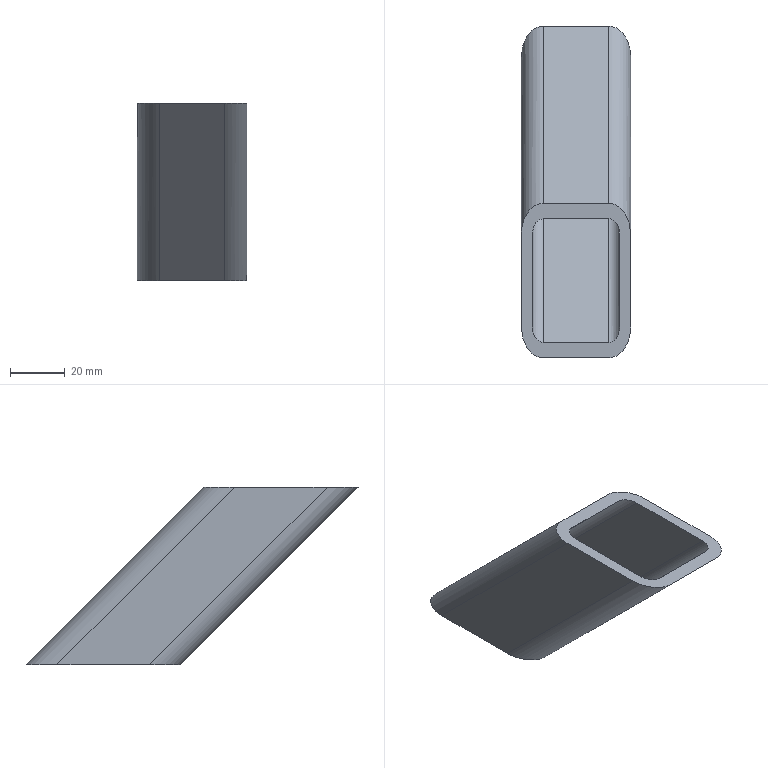Component | SolidWorks | 01-01Chassis-1_01-01-02ChassisWeldment2-1 | 1 solid | 18 faces | box 40 x 121.57 x 65 mm | volume 49161 mm3 | plane 10 | cylinder 8 | commonest cylinder face diameters 16 x4 8 x4 | material Q235
STEP:
#1=COLOUR_RGB('',0.7922,0.8196,0.9333);
#2=FILL_AREA_STYLE_COLOUR('',#1);
#3=FILL_AREA_STYLE('',(#2));
#4=SURFACE_STYLE_FILL_AREA(#3);
#5=SURFACE_SIDE_STYLE('',(#4));
#6=SURFACE_STYLE_USAGE(.BOTH.,#5);
#7=PRESENTATION_STYLE_ASSIGNMENT((#6));
#8=CARTESIAN_POINT('',(11.339,1.575,14.961));
#9=VERTEX_POINT('',#8);
#10=CARTESIAN_POINT('',(12.283,1.575,14.961));
#11=VERTEX_POINT('',#10);
#12=CARTESIAN_POINT('',(12.283,1.575,14.961));
#13=DIRECTION('',(1.,-0.,-0.));
#14=VECTOR('',#13,39.37);
#15=LINE('',#12,#14);
#16=EDGE_CURVE('',#9,#11,#15,.T.);
#17=ORIENTED_EDGE('',*,*,#16,.F.);
#18=CARTESIAN_POINT('',(11.339,-0.9843,17.52));
#19=VERTEX_POINT('',#18);
#20=CARTESIAN_POINT('',(11.339,1.892,14.643));
#21=DIRECTION('',(0.,-0.7071,0.7071));
#22=VECTOR('',#21,39.37);
#23=LINE('',#20,#22);
#24=EDGE_CURVE('',#9,#19,#23,.T.);
#25=ORIENTED_EDGE('',*,*,#24,.T.);
#26=CARTESIAN_POINT('',(12.283,-0.9843,17.52));
#27=VERTEX_POINT('',#26);
#28=CARTESIAN_POINT('',(12.283,-0.9843,17.52));
#29=DIRECTION('',(-1.,0.,0.));
#30=VECTOR('',#29,39.37);
#31=LINE('',#28,#30);
#32=EDGE_CURVE('',#27,#19,#31,.T.);
#33=ORIENTED_EDGE('',*,*,#32,.F.);
#34=CARTESIAN_POINT('',(12.283,1.892,14.643));
#35=DIRECTION('',(0.,-0.7071,0.7071));
#36=VECTOR('',#35,39.37);
#37=LINE('',#34,#36);
#38=EDGE_CURVE('',#11,#27,#37,.T.);
#39=ORIENTED_EDGE('',*,*,#38,.F.);
#40=EDGE_LOOP('',(#17,#25,#33,#39));
#41=FACE_OUTER_BOUND('',#40,.T.);
#42=CARTESIAN_POINT('',(12.283,1.892,14.643));
#43=DIRECTION('',(-0.,-0.7071,-0.7071));
#44=DIRECTION('',(-1.,0.,0.));
#45=AXIS2_PLACEMENT_3D('',#42,#43,#44);
#46=PLANE('',#45);
#47=ADVANCED_FACE('',(#41),#46,.F.);
#48=CARTESIAN_POINT('',(11.024,1.129,14.961));
#49=VERTEX_POINT('',#48);
#50=CARTESIAN_POINT('',(11.024,1.129,14.961));
#51=CARTESIAN_POINT('',(11.024,1.39,14.961));
#52=CARTESIAN_POINT('',(11.154,1.575,14.961));
#53=CARTESIAN_POINT('',(11.339,1.575,14.961));
#54=(BOUNDED_CURVE()B_SPLINE_CURVE(3,(#50,#51,#52,#53),.UNSPECIFIED.,.F.,.F.)B_SPLINE_CURVE_WITH_KNOTS((4,4),(1.571,3.142),.UNSPECIFIED.)CURVE()GEOMETRIC_REPRESENTATION_ITEM()RATIONAL_B_SPLINE_CURVE((1.,0.8047,0.8047,1.))REPRESENTATION_ITEM(''));
#55=EDGE_CURVE('',#49,#9,#54,.T.);
#56=ORIENTED_EDGE('',*,*,#55,.F.);
#57=CARTESIAN_POINT('',(11.024,-1.43,17.52));
#58=VERTEX_POINT('',#57);
#59=CARTESIAN_POINT('',(11.024,1.67,14.42));
#60=DIRECTION('',(0.,-0.7071,0.7071));
#61=VECTOR('',#60,39.37);
#62=LINE('',#59,#61);
#63=EDGE_CURVE('',#49,#58,#62,.T.);
#64=ORIENTED_EDGE('',*,*,#63,.T.);
#65=CARTESIAN_POINT('',(11.339,-0.9843,17.52));
#66=CARTESIAN_POINT('',(11.154,-0.9843,17.52));
#67=CARTESIAN_POINT('',(11.024,-1.169,17.52));
#68=CARTESIAN_POINT('',(11.024,-1.43,17.52));
#69=(BOUNDED_CURVE()B_SPLINE_CURVE(3,(#65,#66,#67,#68),.UNSPECIFIED.,.F.,.F.)B_SPLINE_CURVE_WITH_KNOTS((4,4),(3.142,4.712),.UNSPECIFIED.)CURVE()GEOMETRIC_REPRESENTATION_ITEM()RATIONAL_B_SPLINE_CURVE((1.,0.8047,0.8047,1.))REPRESENTATION_ITEM(''));
#70=EDGE_CURVE('',#19,#58,#69,.T.);
#71=ORIENTED_EDGE('',*,*,#70,.F.);
#72=ORIENTED_EDGE('',*,*,#24,.F.);
#73=EDGE_LOOP('',(#56,#64,#71,#72));
#74=FACE_OUTER_BOUND('',#73,.T.);
#75=CARTESIAN_POINT('',(11.339,1.67,14.42));
#76=DIRECTION('',(0.,-0.7071,0.7071));
#77=DIRECTION('',(-1.,0.,0.));
#78=AXIS2_PLACEMENT_3D('',#75,#76,#77);
#79=CYLINDRICAL_SURFACE('',#78,0.315);
#80=ADVANCED_FACE('',(#74),#79,.T.);
#81=CARTESIAN_POINT('',(11.024,-0.2069,14.961));
#82=VERTEX_POINT('',#81);
#83=CARTESIAN_POINT('',(11.024,2.686,14.961));
#84=DIRECTION('',(0.,1.,0.));
#85=VECTOR('',#84,39.37);
#86=LINE('',#83,#85);
#87=EDGE_CURVE('',#82,#49,#86,.T.);
#88=ORIENTED_EDGE('',*,*,#87,.F.);
#89=CARTESIAN_POINT('',(11.024,-2.766,17.52));
#90=VERTEX_POINT('',#89);
#91=CARTESIAN_POINT('',(11.024,1.001,13.752));
#92=DIRECTION('',(0.,-0.7071,0.7071));
#93=VECTOR('',#92,39.37);
#94=LINE('',#91,#93);
#95=EDGE_CURVE('',#82,#90,#94,.T.);
#96=ORIENTED_EDGE('',*,*,#95,.T.);
#97=CARTESIAN_POINT('',(11.024,2.686,17.52));
#98=DIRECTION('',(-0.,-1.,-0.));
#99=VECTOR('',#98,39.37);
#100=LINE('',#97,#99);
#101=EDGE_CURVE('',#58,#90,#100,.T.);
#102=ORIENTED_EDGE('',*,*,#101,.F.);
#103=ORIENTED_EDGE('',*,*,#63,.F.);
#104=EDGE_LOOP('',(#88,#96,#102,#103));
#105=FACE_OUTER_BOUND('',#104,.T.);
#106=CARTESIAN_POINT('',(11.024,1.001,13.752));
#107=DIRECTION('',(1.,-0.,-0.));
#108=DIRECTION('',(-0.,-0.7071,-0.7071));
#109=AXIS2_PLACEMENT_3D('',#106,#107,#108);
#110=PLANE('',#109);
#111=ADVANCED_FACE('',(#105),#110,.F.);
#112=CARTESIAN_POINT('',(11.339,-0.6523,14.961));
#113=VERTEX_POINT('',#112);
#114=CARTESIAN_POINT('',(11.339,-0.6523,14.961));
#115=CARTESIAN_POINT('',(11.154,-0.6523,14.961));
#116=CARTESIAN_POINT('',(11.024,-0.4678,14.961));
#117=CARTESIAN_POINT('',(11.024,-0.2069,14.961));
#118=(BOUNDED_CURVE()B_SPLINE_CURVE(3,(#114,#115,#116,#117),.UNSPECIFIED.,.F.,.F.)B_SPLINE_CURVE_WITH_KNOTS((4,4),(0.,1.571),.UNSPECIFIED.)CURVE()GEOMETRIC_REPRESENTATION_ITEM()RATIONAL_B_SPLINE_CURVE((1.,0.8047,0.8047,1.))REPRESENTATION_ITEM(''));
#119=EDGE_CURVE('',#113,#82,#118,.T.);
#120=ORIENTED_EDGE('',*,*,#119,.F.);
#121=CARTESIAN_POINT('',(11.339,-3.211,17.52));
#122=VERTEX_POINT('',#121);
#123=CARTESIAN_POINT('',(11.339,0.7788,13.53));
#124=DIRECTION('',(0.,-0.7071,0.7071));
#125=VECTOR('',#124,39.37);
#126=LINE('',#123,#125);
#127=EDGE_CURVE('',#113,#122,#126,.T.);
#128=ORIENTED_EDGE('',*,*,#127,.T.);
#129=CARTESIAN_POINT('',(11.024,-2.766,17.52));
#130=CARTESIAN_POINT('',(11.024,-3.027,17.52));
#131=CARTESIAN_POINT('',(11.154,-3.211,17.52));
#132=CARTESIAN_POINT('',(11.339,-3.211,17.52));
#133=(BOUNDED_CURVE()B_SPLINE_CURVE(3,(#129,#130,#131,#132),.UNSPECIFIED.,.F.,.F.)B_SPLINE_CURVE_WITH_KNOTS((4,4),(4.712,6.283),.UNSPECIFIED.)CURVE()GEOMETRIC_REPRESENTATION_ITEM()RATIONAL_B_SPLINE_CURVE((1.,0.8047,0.8047,1.))REPRESENTATION_ITEM(''));
#134=EDGE_CURVE('',#90,#122,#133,.T.);
#135=ORIENTED_EDGE('',*,*,#134,.F.);
#136=ORIENTED_EDGE('',*,*,#95,.F.);
#137=EDGE_LOOP('',(#120,#128,#135,#136));
#138=FACE_OUTER_BOUND('',#137,.T.);
#139=CARTESIAN_POINT('',(11.339,1.001,13.752));
#140=DIRECTION('',(0.,-0.7071,0.7071));
#141=DIRECTION('',(-1.,0.,0.));
#142=AXIS2_PLACEMENT_3D('',#139,#140,#141);
#143=CYLINDRICAL_SURFACE('',#142,0.315);
#144=ADVANCED_FACE('',(#138),#143,.T.);
#145=CARTESIAN_POINT('',(12.283,-0.6523,14.961));
#146=VERTEX_POINT('',#145);
#147=CARTESIAN_POINT('',(11.339,-0.6523,14.961));
#148=DIRECTION('',(-1.,0.,0.));
#149=VECTOR('',#148,39.37);
#150=LINE('',#147,#149);
#151=EDGE_CURVE('',#146,#113,#150,.T.);
#152=ORIENTED_EDGE('',*,*,#151,.F.);
#153=CARTESIAN_POINT('',(12.283,-3.211,17.52));
#154=VERTEX_POINT('',#153);
#155=CARTESIAN_POINT('',(12.283,0.7788,13.53));
#156=DIRECTION('',(0.,-0.7071,0.7071));
#157=VECTOR('',#156,39.37);
#158=LINE('',#155,#157);
#159=EDGE_CURVE('',#146,#154,#158,.T.);
#160=ORIENTED_EDGE('',*,*,#159,.T.);
#161=CARTESIAN_POINT('',(11.339,-3.211,17.52));
#162=DIRECTION('',(1.,-0.,-0.));
#163=VECTOR('',#162,39.37);
#164=LINE('',#161,#163);
#165=EDGE_CURVE('',#122,#154,#164,.T.);
#166=ORIENTED_EDGE('',*,*,#165,.F.);
#167=ORIENTED_EDGE('',*,*,#127,.F.);
#168=EDGE_LOOP('',(#152,#160,#166,#167));
#169=FACE_OUTER_BOUND('',#168,.T.);
#170=CARTESIAN_POINT('',(11.339,0.7788,13.53));
#171=DIRECTION('',(0.,0.7071,0.7071));
#172=DIRECTION('',(1.,-0.,-0.));
#173=AXIS2_PLACEMENT_3D('',#170,#171,#172);
#174=PLANE('',#173);
#175=ADVANCED_FACE('',(#169),#174,.F.);
#176=CARTESIAN_POINT('',(12.598,-0.2069,14.961));
#177=VERTEX_POINT('',#176);
#178=CARTESIAN_POINT('',(12.598,-0.2069,14.961));
#179=CARTESIAN_POINT('',(12.598,-0.4678,14.961));
#180=CARTESIAN_POINT('',(12.468,-0.6523,14.961));
#181=CARTESIAN_POINT('',(12.283,-0.6523,14.961));
#182=(BOUNDED_CURVE()B_SPLINE_CURVE(3,(#178,#179,#180,#181),.UNSPECIFIED.,.F.,.F.)B_SPLINE_CURVE_WITH_KNOTS((4,4),(4.712,6.283),.UNSPECIFIED.)CURVE()GEOMETRIC_REPRESENTATION_ITEM()RATIONAL_B_SPLINE_CURVE((1.,0.8047,0.8047,1.))REPRESENTATION_ITEM(''));
#183=EDGE_CURVE('',#177,#146,#182,.T.);
#184=ORIENTED_EDGE('',*,*,#183,.F.);
#185=CARTESIAN_POINT('',(12.598,-2.766,17.52));
#186=VERTEX_POINT('',#185);
#187=CARTESIAN_POINT('',(12.598,1.001,13.752));
#188=DIRECTION('',(0.,-0.7071,0.7071));
#189=VECTOR('',#188,39.37);
#190=LINE('',#187,#189);
#191=EDGE_CURVE('',#177,#186,#190,.T.);
#192=ORIENTED_EDGE('',*,*,#191,.T.);
#193=CARTESIAN_POINT('',(12.283,-3.211,17.52));
#194=CARTESIAN_POINT('',(12.468,-3.211,17.52));
#195=CARTESIAN_POINT('',(12.598,-3.027,17.52));
#196=CARTESIAN_POINT('',(12.598,-2.766,17.52));
#197=(BOUNDED_CURVE()B_SPLINE_CURVE(3,(#193,#194,#195,#196),.UNSPECIFIED.,.F.,.F.)B_SPLINE_CURVE_WITH_KNOTS((4,4),(0.,1.571),.UNSPECIFIED.)CURVE()GEOMETRIC_REPRESENTATION_ITEM()RATIONAL_B_SPLINE_CURVE((1.,0.8047,0.8047,1.))REPRESENTATION_ITEM(''));
#198=EDGE_CURVE('',#154,#186,#197,.T.);
#199=ORIENTED_EDGE('',*,*,#198,.F.);
#200=ORIENTED_EDGE('',*,*,#159,.F.);
#201=EDGE_LOOP('',(#184,#192,#199,#200));
#202=FACE_OUTER_BOUND('',#201,.T.);
#203=CARTESIAN_POINT('',(12.283,1.001,13.752));
#204=DIRECTION('',(0.,-0.7071,0.7071));
#205=DIRECTION('',(-1.,0.,0.));
#206=AXIS2_PLACEMENT_3D('',#203,#204,#205);
#207=CYLINDRICAL_SURFACE('',#206,0.315);
#208=ADVANCED_FACE('',(#202),#207,.T.);
#209=CARTESIAN_POINT('',(12.598,1.129,14.961));
#210=VERTEX_POINT('',#209);
#211=CARTESIAN_POINT('',(12.598,2.686,14.961));
#212=DIRECTION('',(0.,1.,0.));
#213=VECTOR('',#212,39.37);
#214=LINE('',#211,#213);
#215=EDGE_CURVE('',#177,#210,#214,.T.);
#216=ORIENTED_EDGE('',*,*,#215,.T.);
#217=CARTESIAN_POINT('',(12.598,-1.43,17.52));
#218=VERTEX_POINT('',#217);
#219=CARTESIAN_POINT('',(12.598,1.67,14.42));
#220=DIRECTION('',(0.,-0.7071,0.7071));
#221=VECTOR('',#220,39.37);
#222=LINE('',#219,#221);
#223=EDGE_CURVE('',#210,#218,#222,.T.);
#224=ORIENTED_EDGE('',*,*,#223,.T.);
#225=CARTESIAN_POINT('',(12.598,2.686,17.52));
#226=DIRECTION('',(-0.,-1.,-0.));
#227=VECTOR('',#226,39.37);
#228=LINE('',#225,#227);
#229=EDGE_CURVE('',#218,#186,#228,.T.);
#230=ORIENTED_EDGE('',*,*,#229,.T.);
#231=ORIENTED_EDGE('',*,*,#191,.F.);
#232=EDGE_LOOP('',(#216,#224,#230,#231));
#233=FACE_OUTER_BOUND('',#232,.T.);
#234=CARTESIAN_POINT('',(12.598,1.67,14.42));
#235=DIRECTION('',(-1.,0.,0.));
#236=DIRECTION('',(0.,0.7071,0.7071));
#237=AXIS2_PLACEMENT_3D('',#234,#235,#236);
#238=PLANE('',#237);
#239=ADVANCED_FACE('',(#233),#238,.F.);
#240=CARTESIAN_POINT('',(12.283,1.575,14.961));
#241=CARTESIAN_POINT('',(12.468,1.575,14.961));
#242=CARTESIAN_POINT('',(12.598,1.39,14.961));
#243=CARTESIAN_POINT('',(12.598,1.129,14.961));
#244=(BOUNDED_CURVE()B_SPLINE_CURVE(3,(#240,#241,#242,#243),.UNSPECIFIED.,.F.,.F.)B_SPLINE_CURVE_WITH_KNOTS((4,4),(3.142,4.712),.UNSPECIFIED.)CURVE()GEOMETRIC_REPRESENTATION_ITEM()RATIONAL_B_SPLINE_CURVE((1.,0.8047,0.8047,1.))REPRESENTATION_ITEM(''));
#245=EDGE_CURVE('',#11,#210,#244,.T.);
#246=ORIENTED_EDGE('',*,*,#245,.F.);
#247=ORIENTED_EDGE('',*,*,#38,.T.);
#248=CARTESIAN_POINT('',(12.598,-1.43,17.52));
#249=CARTESIAN_POINT('',(12.598,-1.169,17.52));
#250=CARTESIAN_POINT('',(12.468,-0.9843,17.52));
#251=CARTESIAN_POINT('',(12.283,-0.9843,17.52));
#252=(BOUNDED_CURVE()B_SPLINE_CURVE(3,(#248,#249,#250,#251),.UNSPECIFIED.,.F.,.F.)B_SPLINE_CURVE_WITH_KNOTS((4,4),(1.571,3.142),.UNSPECIFIED.)CURVE()GEOMETRIC_REPRESENTATION_ITEM()RATIONAL_B_SPLINE_CURVE((1.,0.8047,0.8047,1.))REPRESENTATION_ITEM(''));
#253=EDGE_CURVE('',#218,#27,#252,.T.);
#254=ORIENTED_EDGE('',*,*,#253,.F.);
#255=ORIENTED_EDGE('',*,*,#223,.F.);
#256=EDGE_LOOP('',(#246,#247,#254,#255));
#257=FACE_OUTER_BOUND('',#256,.T.);
#258=CARTESIAN_POINT('',(12.283,1.67,14.42));
#259=DIRECTION('',(0.,-0.7071,0.7071));
#260=DIRECTION('',(-1.,0.,0.));
#261=AXIS2_PLACEMENT_3D('',#258,#259,#260);
#262=CYLINDRICAL_SURFACE('',#261,0.315);
#263=ADVANCED_FACE('',(#257),#262,.T.);
#264=CARTESIAN_POINT('',(11.339,-2.989,17.52));
#265=VERTEX_POINT('',#264);
#266=CARTESIAN_POINT('',(12.283,-2.989,17.52));
#267=VERTEX_POINT('',#266);
#268=CARTESIAN_POINT('',(11.339,-2.989,17.52));
#269=DIRECTION('',(1.,-0.,-0.));
#270=VECTOR('',#269,39.37);
#271=LINE('',#268,#270);
#272=EDGE_CURVE('',#265,#267,#271,.T.);
#273=ORIENTED_EDGE('',*,*,#272,.F.);
#274=CARTESIAN_POINT('',(11.181,-2.766,17.52));
#275=VERTEX_POINT('',#274);
#276=CARTESIAN_POINT('',(11.181,-2.766,17.52));
#277=CARTESIAN_POINT('',(11.181,-2.896,17.52));
#278=CARTESIAN_POINT('',(11.246,-2.989,17.52));
#279=CARTESIAN_POINT('',(11.339,-2.989,17.52));
#280=(BOUNDED_CURVE()B_SPLINE_CURVE(3,(#276,#277,#278,#279),.UNSPECIFIED.,.F.,.F.)B_SPLINE_CURVE_WITH_KNOTS((4,4),(4.712,6.283),.UNSPECIFIED.)CURVE()GEOMETRIC_REPRESENTATION_ITEM()RATIONAL_B_SPLINE_CURVE((1.,0.8047,0.8047,1.))REPRESENTATION_ITEM(''));
#281=EDGE_CURVE('',#275,#265,#280,.T.);
#282=ORIENTED_EDGE('',*,*,#281,.F.);
#283=CARTESIAN_POINT('',(11.181,-1.43,17.52));
#284=VERTEX_POINT('',#283);
#285=CARTESIAN_POINT('',(11.181,1.001,17.52));
#286=DIRECTION('',(-0.,-1.,-0.));
#287=VECTOR('',#286,39.37);
#288=LINE('',#285,#287);
#289=EDGE_CURVE('',#284,#275,#288,.T.);
#290=ORIENTED_EDGE('',*,*,#289,.F.);
#291=CARTESIAN_POINT('',(11.339,-1.207,17.52));
#292=VERTEX_POINT('',#291);
#293=CARTESIAN_POINT('',(11.339,-1.207,17.52));
#294=CARTESIAN_POINT('',(11.246,-1.207,17.52));
#295=CARTESIAN_POINT('',(11.181,-1.299,17.52));
#296=CARTESIAN_POINT('',(11.181,-1.43,17.52));
#297=(BOUNDED_CURVE()B_SPLINE_CURVE(3,(#293,#294,#295,#296),.UNSPECIFIED.,.F.,.F.)B_SPLINE_CURVE_WITH_KNOTS((4,4),(3.142,4.712),.UNSPECIFIED.)CURVE()GEOMETRIC_REPRESENTATION_ITEM()RATIONAL_B_SPLINE_CURVE((1.,0.8047,0.8047,1.))REPRESENTATION_ITEM(''));
#298=EDGE_CURVE('',#292,#284,#297,.T.);
#299=ORIENTED_EDGE('',*,*,#298,.F.);
#300=CARTESIAN_POINT('',(12.283,-1.207,17.52));
#301=VERTEX_POINT('',#300);
#302=CARTESIAN_POINT('',(12.283,-1.207,17.52));
#303=DIRECTION('',(-1.,0.,0.));
#304=VECTOR('',#303,39.37);
#305=LINE('',#302,#304);
#306=EDGE_CURVE('',#301,#292,#305,.T.);
#307=ORIENTED_EDGE('',*,*,#306,.F.);
#308=CARTESIAN_POINT('',(12.441,-1.43,17.52));
#309=VERTEX_POINT('',#308);
#310=CARTESIAN_POINT('',(12.441,-1.43,17.52));
#311=CARTESIAN_POINT('',(12.441,-1.299,17.52));
#312=CARTESIAN_POINT('',(12.376,-1.207,17.52));
#313=CARTESIAN_POINT('',(12.283,-1.207,17.52));
#314=(BOUNDED_CURVE()B_SPLINE_CURVE(3,(#310,#311,#312,#313),.UNSPECIFIED.,.F.,.F.)B_SPLINE_CURVE_WITH_KNOTS((4,4),(1.571,3.142),.UNSPECIFIED.)CURVE()GEOMETRIC_REPRESENTATION_ITEM()RATIONAL_B_SPLINE_CURVE((1.,0.8047,0.8047,1.))REPRESENTATION_ITEM(''));
#315=EDGE_CURVE('',#309,#301,#314,.T.);
#316=ORIENTED_EDGE('',*,*,#315,.F.);
#317=CARTESIAN_POINT('',(12.441,-2.766,17.52));
#318=VERTEX_POINT('',#317);
#319=CARTESIAN_POINT('',(12.441,1.67,17.52));
#320=DIRECTION('',(0.,1.,0.));
#321=VECTOR('',#320,39.37);
#322=LINE('',#319,#321);
#323=EDGE_CURVE('',#318,#309,#322,.T.);
#324=ORIENTED_EDGE('',*,*,#323,.F.);
#325=CARTESIAN_POINT('',(12.283,-2.989,17.52));
#326=CARTESIAN_POINT('',(12.376,-2.989,17.52));
#327=CARTESIAN_POINT('',(12.441,-2.896,17.52));
#328=CARTESIAN_POINT('',(12.441,-2.766,17.52));
#329=(BOUNDED_CURVE()B_SPLINE_CURVE(3,(#325,#326,#327,#328),.UNSPECIFIED.,.F.,.F.)B_SPLINE_CURVE_WITH_KNOTS((4,4),(0.,1.571),.UNSPECIFIED.)CURVE()GEOMETRIC_REPRESENTATION_ITEM()RATIONAL_B_SPLINE_CURVE((1.,0.8047,0.8047,1.))REPRESENTATION_ITEM(''));
#330=EDGE_CURVE('',#267,#318,#329,.T.);
#331=ORIENTED_EDGE('',*,*,#330,.F.);
#332=EDGE_LOOP('',(#273,#282,#290,#299,#307,#316,#324,#331));
#333=FACE_BOUND('',#332,.T.);
#334=ORIENTED_EDGE('',*,*,#198,.T.);
#335=ORIENTED_EDGE('',*,*,#229,.F.);
#336=ORIENTED_EDGE('',*,*,#253,.T.);
#337=ORIENTED_EDGE('',*,*,#32,.T.);
#338=ORIENTED_EDGE('',*,*,#70,.T.);
#339=ORIENTED_EDGE('',*,*,#101,.T.);
#340=ORIENTED_EDGE('',*,*,#134,.T.);
#341=ORIENTED_EDGE('',*,*,#165,.T.);
#342=EDGE_LOOP('',(#334,#335,#336,#337,#338,#339,#340,#341));
#343=FACE_OUTER_BOUND('',#342,.T.);
#344=CARTESIAN_POINT('',(11.024,2.686,17.52));
#345=DIRECTION('',(0.,-0.,1.));
#346=DIRECTION('',(-0.,-1.,-0.));
#347=AXIS2_PLACEMENT_3D('',#344,#345,#346);
#348=PLANE('',#347);
#349=ADVANCED_FACE('',(#333,#343),#348,.T.);
#350=CARTESIAN_POINT('',(12.441,1.129,14.961));
#351=VERTEX_POINT('',#350);
#352=CARTESIAN_POINT('',(12.441,-0.2069,14.961));
#353=VERTEX_POINT('',#352);
#354=CARTESIAN_POINT('',(12.441,1.67,14.961));
#355=DIRECTION('',(-0.,-1.,-0.));
#356=VECTOR('',#355,39.37);
#357=LINE('',#354,#356);
#358=EDGE_CURVE('',#351,#353,#357,.T.);
#359=ORIENTED_EDGE('',*,*,#358,.F.);
#360=CARTESIAN_POINT('',(12.283,1.352,14.961));
#361=VERTEX_POINT('',#360);
#362=CARTESIAN_POINT('',(12.283,1.352,14.961));
#363=CARTESIAN_POINT('',(12.376,1.352,14.961));
#364=CARTESIAN_POINT('',(12.441,1.26,14.961));
#365=CARTESIAN_POINT('',(12.441,1.129,14.961));
#366=(BOUNDED_CURVE()B_SPLINE_CURVE(3,(#362,#363,#364,#365),.UNSPECIFIED.,.F.,.F.)B_SPLINE_CURVE_WITH_KNOTS((4,4),(3.142,4.712),.UNSPECIFIED.)CURVE()GEOMETRIC_REPRESENTATION_ITEM()RATIONAL_B_SPLINE_CURVE((1.,0.8047,0.8047,1.))REPRESENTATION_ITEM(''));
#367=EDGE_CURVE('',#361,#351,#366,.T.);
#368=ORIENTED_EDGE('',*,*,#367,.F.);
#369=CARTESIAN_POINT('',(11.339,1.352,14.961));
#370=VERTEX_POINT('',#369);
#371=CARTESIAN_POINT('',(12.283,1.352,14.961));
#372=DIRECTION('',(1.,-0.,-0.));
#373=VECTOR('',#372,39.37);
#374=LINE('',#371,#373);
#375=EDGE_CURVE('',#370,#361,#374,.T.);
#376=ORIENTED_EDGE('',*,*,#375,.F.);
#377=CARTESIAN_POINT('',(11.181,1.129,14.961));
#378=VERTEX_POINT('',#377);
#379=CARTESIAN_POINT('',(11.181,1.129,14.961));
#380=CARTESIAN_POINT('',(11.181,1.26,14.961));
#381=CARTESIAN_POINT('',(11.246,1.352,14.961));
#382=CARTESIAN_POINT('',(11.339,1.352,14.961));
#383=(BOUNDED_CURVE()B_SPLINE_CURVE(3,(#379,#380,#381,#382),.UNSPECIFIED.,.F.,.F.)B_SPLINE_CURVE_WITH_KNOTS((4,4),(1.571,3.142),.UNSPECIFIED.)CURVE()GEOMETRIC_REPRESENTATION_ITEM()RATIONAL_B_SPLINE_CURVE((1.,0.8047,0.8047,1.))REPRESENTATION_ITEM(''));
#384=EDGE_CURVE('',#378,#370,#383,.T.);
#385=ORIENTED_EDGE('',*,*,#384,.F.);
#386=CARTESIAN_POINT('',(11.181,-0.2069,14.961));
#387=VERTEX_POINT('',#386);
#388=CARTESIAN_POINT('',(11.181,1.001,14.961));
#389=DIRECTION('',(0.,1.,0.));
#390=VECTOR('',#389,39.37);
#391=LINE('',#388,#390);
#392=EDGE_CURVE('',#387,#378,#391,.T.);
#393=ORIENTED_EDGE('',*,*,#392,.F.);
#394=CARTESIAN_POINT('',(11.339,-0.4296,14.961));
#395=VERTEX_POINT('',#394);
#396=CARTESIAN_POINT('',(11.339,-0.4296,14.961));
#397=CARTESIAN_POINT('',(11.246,-0.4296,14.961));
#398=CARTESIAN_POINT('',(11.181,-0.3373,14.961));
#399=CARTESIAN_POINT('',(11.181,-0.2069,14.961));
#400=(BOUNDED_CURVE()B_SPLINE_CURVE(3,(#396,#397,#398,#399),.UNSPECIFIED.,.F.,.T.)B_SPLINE_CURVE_WITH_KNOTS((4,4),(0.,1.571),.UNSPECIFIED.)CURVE()GEOMETRIC_REPRESENTATION_ITEM()RATIONAL_B_SPLINE_CURVE((1.,0.8047,0.8047,1.))REPRESENTATION_ITEM(''));
#401=EDGE_CURVE('',#395,#387,#400,.T.);
#402=ORIENTED_EDGE('',*,*,#401,.F.);
#403=CARTESIAN_POINT('',(12.283,-0.4296,14.961));
#404=VERTEX_POINT('',#403);
#405=CARTESIAN_POINT('',(11.339,-0.4296,14.961));
#406=DIRECTION('',(-1.,0.,0.));
#407=VECTOR('',#406,39.37);
#408=LINE('',#405,#407);
#409=EDGE_CURVE('',#404,#395,#408,.T.);
#410=ORIENTED_EDGE('',*,*,#409,.F.);
#411=CARTESIAN_POINT('',(12.441,-0.2069,14.961));
#412=CARTESIAN_POINT('',(12.441,-0.3373,14.961));
#413=CARTESIAN_POINT('',(12.376,-0.4296,14.961));
#414=CARTESIAN_POINT('',(12.283,-0.4296,14.961));
#415=(BOUNDED_CURVE()B_SPLINE_CURVE(3,(#411,#412,#413,#414),.UNSPECIFIED.,.F.,.F.)B_SPLINE_CURVE_WITH_KNOTS((4,4),(4.712,6.283),.UNSPECIFIED.)CURVE()GEOMETRIC_REPRESENTATION_ITEM()RATIONAL_B_SPLINE_CURVE((1.,0.8047,0.8047,1.))REPRESENTATION_ITEM(''));
#416=EDGE_CURVE('',#353,#404,#415,.T.);
#417=ORIENTED_EDGE('',*,*,#416,.F.);
#418=EDGE_LOOP('',(#359,#368,#376,#385,#393,#402,#410,#417));
#419=FACE_BOUND('',#418,.T.);
#420=ORIENTED_EDGE('',*,*,#183,.T.);
#421=ORIENTED_EDGE('',*,*,#151,.T.);
#422=ORIENTED_EDGE('',*,*,#119,.T.);
#423=ORIENTED_EDGE('',*,*,#87,.T.);
#424=ORIENTED_EDGE('',*,*,#55,.T.);
#425=ORIENTED_EDGE('',*,*,#16,.T.);
#426=ORIENTED_EDGE('',*,*,#245,.T.);
#427=ORIENTED_EDGE('',*,*,#215,.F.);
#428=EDGE_LOOP('',(#420,#421,#422,#423,#424,#425,#426,#427));
#429=FACE_OUTER_BOUND('',#428,.T.);
#430=CARTESIAN_POINT('',(11.024,2.686,14.961));
#431=DIRECTION('',(-0.,0.,-1.));
#432=DIRECTION('',(0.,1.,0.));
#433=AXIS2_PLACEMENT_3D('',#430,#431,#432);
#434=PLANE('',#433);
#435=ADVANCED_FACE('',(#419,#429),#434,.T.);
#436=CARTESIAN_POINT('',(12.441,1.001,13.752));
#437=DIRECTION('',(0.,-0.7071,0.7071));
#438=VECTOR('',#437,39.37);
#439=LINE('',#436,#438);
#440=EDGE_CURVE('',#353,#318,#439,.T.);
#441=ORIENTED_EDGE('',*,*,#440,.F.);
#442=ORIENTED_EDGE('',*,*,#416,.T.);
#443=CARTESIAN_POINT('',(12.283,0.8901,13.641));
#444=DIRECTION('',(0.,-0.7071,0.7071));
#445=VECTOR('',#444,39.37);
#446=LINE('',#443,#445);
#447=EDGE_CURVE('',#404,#267,#446,.T.);
#448=ORIENTED_EDGE('',*,*,#447,.T.);
#449=ORIENTED_EDGE('',*,*,#330,.T.);
#450=EDGE_LOOP('',(#441,#442,#448,#449));
#451=FACE_OUTER_BOUND('',#450,.T.);
#452=CARTESIAN_POINT('',(12.283,1.001,13.752));
#453=DIRECTION('',(0.,-0.7071,0.7071));
#454=DIRECTION('',(-1.,0.,0.));
#455=AXIS2_PLACEMENT_3D('',#452,#453,#454);
#456=CYLINDRICAL_SURFACE('',#455,0.1575);
#457=ADVANCED_FACE('',(#451),#456,.F.);
#458=CARTESIAN_POINT('',(12.441,1.67,14.42));
#459=DIRECTION('',(0.,-0.7071,0.7071));
#460=VECTOR('',#459,39.37);
#461=LINE('',#458,#460);
#462=EDGE_CURVE('',#351,#309,#461,.T.);
#463=ORIENTED_EDGE('',*,*,#462,.F.);
#464=ORIENTED_EDGE('',*,*,#358,.T.);
#465=ORIENTED_EDGE('',*,*,#440,.T.);
#466=ORIENTED_EDGE('',*,*,#323,.T.);
#467=EDGE_LOOP('',(#463,#464,#465,#466));
#468=FACE_OUTER_BOUND('',#467,.T.);
#469=CARTESIAN_POINT('',(12.441,1.67,14.42));
#470=DIRECTION('',(-1.,0.,0.));
#471=DIRECTION('',(0.,0.7071,0.7071));
#472=AXIS2_PLACEMENT_3D('',#469,#470,#471);
#473=PLANE('',#472);
#474=ADVANCED_FACE('',(#468),#473,.T.);
#475=CARTESIAN_POINT('',(12.283,1.781,14.532));
#476=DIRECTION('',(0.,-0.7071,0.7071));
#477=VECTOR('',#476,39.37);
#478=LINE('',#475,#477);
#479=EDGE_CURVE('',#361,#301,#478,.T.);
#480=ORIENTED_EDGE('',*,*,#479,.F.);
#481=ORIENTED_EDGE('',*,*,#367,.T.);
#482=ORIENTED_EDGE('',*,*,#462,.T.);
#483=ORIENTED_EDGE('',*,*,#315,.T.);
#484=EDGE_LOOP('',(#480,#481,#482,#483));
#485=FACE_OUTER_BOUND('',#484,.T.);
#486=CARTESIAN_POINT('',(12.283,1.67,14.42));
#487=DIRECTION('',(0.,-0.7071,0.7071));
#488=DIRECTION('',(-1.,0.,0.));
#489=AXIS2_PLACEMENT_3D('',#486,#487,#488);
#490=CYLINDRICAL_SURFACE('',#489,0.1575);
#491=ADVANCED_FACE('',(#485),#490,.F.);
#492=CARTESIAN_POINT('',(11.339,1.781,14.532));
#493=DIRECTION('',(0.,-0.7071,0.7071));
#494=VECTOR('',#493,39.37);
#495=LINE('',#492,#494);
#496=EDGE_CURVE('',#370,#292,#495,.T.);
#497=ORIENTED_EDGE('',*,*,#496,.F.);
#498=ORIENTED_EDGE('',*,*,#375,.T.);
#499=ORIENTED_EDGE('',*,*,#479,.T.);
#500=ORIENTED_EDGE('',*,*,#306,.T.);
#501=EDGE_LOOP('',(#497,#498,#499,#500));
#502=FACE_OUTER_BOUND('',#501,.T.);
#503=CARTESIAN_POINT('',(12.283,1.781,14.532));
#504=DIRECTION('',(-0.,-0.7071,-0.7071));
#505=DIRECTION('',(-1.,0.,0.));
#506=AXIS2_PLACEMENT_3D('',#503,#504,#505);
#507=PLANE('',#506);
#508=ADVANCED_FACE('',(#502),#507,.T.);
#509=CARTESIAN_POINT('',(11.181,1.67,14.42));
#510=DIRECTION('',(0.,-0.7071,0.7071));
#511=VECTOR('',#510,39.37);
#512=LINE('',#509,#511);
#513=EDGE_CURVE('',#378,#284,#512,.T.);
#514=ORIENTED_EDGE('',*,*,#513,.F.);
#515=ORIENTED_EDGE('',*,*,#384,.T.);
#516=ORIENTED_EDGE('',*,*,#496,.T.);
#517=ORIENTED_EDGE('',*,*,#298,.T.);
#518=EDGE_LOOP('',(#514,#515,#516,#517));
#519=FACE_OUTER_BOUND('',#518,.T.);
#520=CARTESIAN_POINT('',(11.339,1.67,14.42));
#521=DIRECTION('',(0.,-0.7071,0.7071));
#522=DIRECTION('',(-1.,0.,0.));
#523=AXIS2_PLACEMENT_3D('',#520,#521,#522);
#524=CYLINDRICAL_SURFACE('',#523,0.1575);
#525=ADVANCED_FACE('',(#519),#524,.F.);
#526=CARTESIAN_POINT('',(11.181,1.001,13.752));
#527=DIRECTION('',(0.,-0.7071,0.7071));
#528=VECTOR('',#527,39.37);
#529=LINE('',#526,#528);
#530=EDGE_CURVE('',#387,#275,#529,.T.);
#531=ORIENTED_EDGE('',*,*,#530,.F.);
#532=ORIENTED_EDGE('',*,*,#392,.T.);
#533=ORIENTED_EDGE('',*,*,#513,.T.);
#534=ORIENTED_EDGE('',*,*,#289,.T.);
#535=EDGE_LOOP('',(#531,#532,#533,#534));
#536=FACE_OUTER_BOUND('',#535,.T.);
#537=CARTESIAN_POINT('',(11.181,1.001,13.752));
#538=DIRECTION('',(1.,-0.,-0.));
#539=DIRECTION('',(-0.,-0.7071,-0.7071));
#540=AXIS2_PLACEMENT_3D('',#537,#538,#539);
#541=PLANE('',#540);
#542=ADVANCED_FACE('',(#536),#541,.T.);
#543=CARTESIAN_POINT('',(11.339,0.8901,13.641));
#544=DIRECTION('',(0.,-0.7071,0.7071));
#545=VECTOR('',#544,39.37);
#546=LINE('',#543,#545);
#547=EDGE_CURVE('',#395,#265,#546,.T.);
#548=ORIENTED_EDGE('',*,*,#547,.F.);
#549=ORIENTED_EDGE('',*,*,#401,.T.);
#550=ORIENTED_EDGE('',*,*,#530,.T.);
#551=ORIENTED_EDGE('',*,*,#281,.T.);
#552=EDGE_LOOP('',(#548,#549,#550,#551));
#553=FACE_OUTER_BOUND('',#552,.T.);
#554=CARTESIAN_POINT('',(11.339,1.001,13.752));
#555=DIRECTION('',(0.,-0.7071,0.7071));
#556=DIRECTION('',(-1.,0.,0.));
#557=AXIS2_PLACEMENT_3D('',#554,#555,#556);
#558=CYLINDRICAL_SURFACE('',#557,0.1575);
#559=ADVANCED_FACE('',(#553),#558,.F.);
#560=ORIENTED_EDGE('',*,*,#447,.F.);
#561=ORIENTED_EDGE('',*,*,#409,.T.);
#562=ORIENTED_EDGE('',*,*,#547,.T.);
#563=ORIENTED_EDGE('',*,*,#272,.T.);
#564=EDGE_LOOP('',(#560,#561,#562,#563));
#565=FACE_OUTER_BOUND('',#564,.T.);
#566=CARTESIAN_POINT('',(11.339,0.8901,13.641));
#567=DIRECTION('',(0.,0.7071,0.7071));
#568=DIRECTION('',(1.,-0.,-0.));
#569=AXIS2_PLACEMENT_3D('',#566,#567,#568);
#570=PLANE('',#569);
#571=ADVANCED_FACE('',(#565),#570,.T.);
#572=CLOSED_SHELL('',(#47,#80,#111,#144,#175,#208,#239,#263,#349,#435,#457,#474,#491,#508,#525,#542,#559,#571));
#573=MANIFOLD_SOLID_BREP('',#572);
#574=STYLED_ITEM('',(#7),#573);
#575=PRESENTATION_LAYER_ASSIGNMENT('','',(#574));
#576=(LENGTH_UNIT()NAMED_UNIT(*)SI_UNIT($,.METRE.));
#577=LENGTH_MEASURE_WITH_UNIT(LENGTH_MEASURE(0.0254),#576);
#578=DIMENSIONAL_EXPONENTS(1.,0.,0.,0.,0.,0.,0.);
#579=(CONVERSION_BASED_UNIT('',#577)LENGTH_UNIT()NAMED_UNIT(#578));
#580=UNCERTAINTY_MEASURE_WITH_UNIT(LENGTH_MEASURE(0.00001),#579,'','');
#581=(NAMED_UNIT(*)PLANE_ANGLE_UNIT()SI_UNIT($,.RADIAN.));
#582=(NAMED_UNIT(*)SI_UNIT($,.STERADIAN.)SOLID_ANGLE_UNIT());
#583=(GEOMETRIC_REPRESENTATION_CONTEXT(3)GLOBAL_UNCERTAINTY_ASSIGNED_CONTEXT((#580))GLOBAL_UNIT_ASSIGNED_CONTEXT((#579,#581,#582))REPRESENTATION_CONTEXT('',''));
#584=MECHANICAL_DESIGN_GEOMETRIC_PRESENTATION_REPRESENTATION('',(#574),#583);
#585=CARTESIAN_POINT('',(0.,0.,0.));
#586=DIRECTION('',(0.,0.,1.));
#587=DIRECTION('',(1.,0.,0.));
#588=AXIS2_PLACEMENT_3D('',#585,#586,#587);
#589=(LENGTH_UNIT()NAMED_UNIT(*)SI_UNIT($,.METRE.));
#590=LENGTH_MEASURE_WITH_UNIT(LENGTH_MEASURE(0.0254),#589);
#591=DIMENSIONAL_EXPONENTS(1.,0.,0.,0.,0.,0.,0.);
#592=(CONVERSION_BASED_UNIT('',#590)LENGTH_UNIT()NAMED_UNIT(#591));
#593=UNCERTAINTY_MEASURE_WITH_UNIT(LENGTH_MEASURE(0.00001),#592,'','');
#594=(NAMED_UNIT(*)PLANE_ANGLE_UNIT()SI_UNIT($,.RADIAN.));
#595=(NAMED_UNIT(*)SI_UNIT($,.STERADIAN.)SOLID_ANGLE_UNIT());
#596=(GEOMETRIC_REPRESENTATION_CONTEXT(3)GLOBAL_UNCERTAINTY_ASSIGNED_CONTEXT((#593))GLOBAL_UNIT_ASSIGNED_CONTEXT((#592,#594,#595))REPRESENTATION_CONTEXT('',''));
#597=ADVANCED_BREP_SHAPE_REPRESENTATION('',(#573,#588),#596);